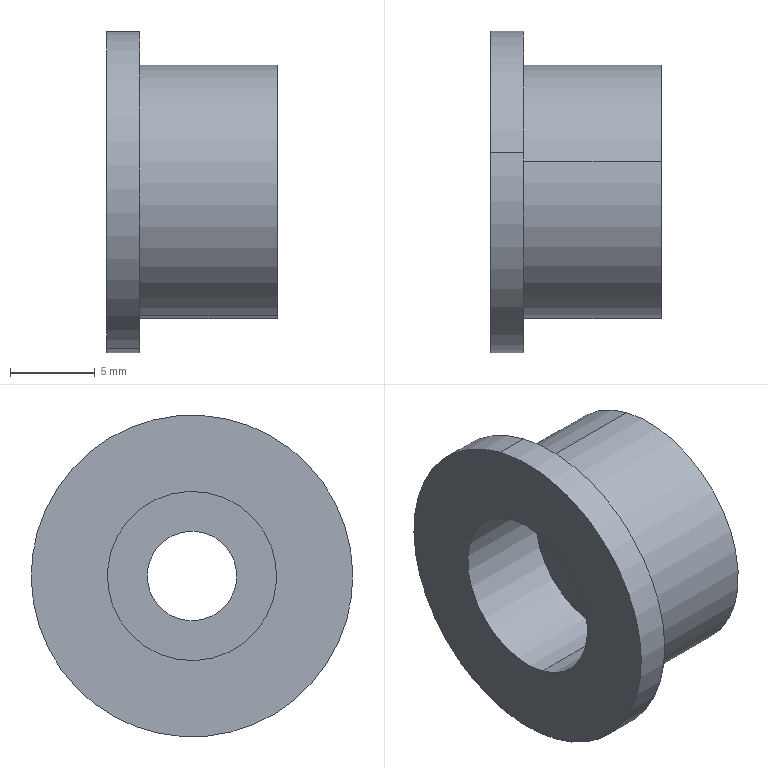Component | SolidWorks | NewDieSet-1_PinDiameter15-3 | 1 solid | 12 faces | box 10.1 x 19 x 19 mm | volume 1448 mm3 | cylinder 8 | plane 4 | commonest cylinder face diameters 10 x2 5.3 x2 19 x2 15 x2
build123d program:
from build123d import *

# Parameters (mm, degrees)
SKETCH1_R                                            = 6
BOSS_EXTRUDE1_DEPTH                                  = 11
SKETCH2_R                                            = 7.5
BOSS_EXTRUDE2_DEPTH                                  = 10.1
SKETCH3_R                                            = 9.5
BOSS_EXTRUDE3_DEPTH                                  = 1.95
HOLE_SIZE_ACCORDING_TO_HEXAGON_SOCKET_HE_D           = 5.3
HOLE_SIZE_ACCORDING_TO_HEXAGON_SOCKET_HE_CBORE_D     = 10
HOLE_SIZE_ACCORDING_TO_HEXAGON_SOCKET_HE_CBORE_DEPTH = 5.7
SKETCH6_R                                            = 6
CUT_EXTRUDE1_DEPTH                                   = 11


with BuildPart() as part:
    # Sketch1 → Boss-Extrude1 (new body)
    with BuildSketch(Plane.XY):
        Circle(SKETCH1_R)
    extrude(amount=BOSS_EXTRUDE1_DEPTH)

    # Sketch2 → Boss-Extrude2 (add)
    with BuildSketch(Plane.XY.offset(11)):
        Circle(SKETCH2_R)
    extrude(amount=BOSS_EXTRUDE2_DEPTH)

    # Sketch3 → Boss-Extrude3 (add)
    with BuildSketch(Plane.XY.offset(21.1)):
        Circle(SKETCH3_R)
    extrude(amount=-BOSS_EXTRUDE3_DEPTH)

    # Hole Size_According to_Hexagon Socket He (through all)
    with Locations(Plane.XY.offset(21.1)):
        with Locations((0, 0)):
            CounterBoreHole(HOLE_SIZE_ACCORDING_TO_HEXAGON_SOCKET_HE_D / 2, HOLE_SIZE_ACCORDING_TO_HEXAGON_SOCKET_HE_CBORE_D / 2, HOLE_SIZE_ACCORDING_TO_HEXAGON_SOCKET_HE_CBORE_DEPTH)

    # Sketch6 → Cut-Extrude1 (cut)
    with BuildSketch(Plane(origin=(0, 0, 0), x_dir=(-1, 0, 0), z_dir=(0, 0, -1))):
        Circle(SKETCH6_R)
    extrude(amount=-CUT_EXTRUDE1_DEPTH, mode=Mode.SUBTRACT)


solid = part.part

# Placed as in the assembly
solid = solid.moved(Location((-245.746, 117.427, 218), (0, -90, 0)))
STEP:
#1=COLOUR_RGB('',0.7922,0.8196,0.9333);
#2=FILL_AREA_STYLE_COLOUR('',#1);
#3=FILL_AREA_STYLE('',(#2));
#4=SURFACE_STYLE_FILL_AREA(#3);
#5=SURFACE_SIDE_STYLE('',(#4));
#6=SURFACE_STYLE_USAGE(.BOTH.,#5);
#7=PRESENTATION_STYLE_ASSIGNMENT((#6));
#8=CARTESIAN_POINT('',(-10.281,4.575,8.392));
#9=VERTEX_POINT('',#8);
#10=CARTESIAN_POINT('',(-10.281,4.671,8.774));
#11=VERTEX_POINT('',#10);
#12=CARTESIAN_POINT('',(-10.281,4.623,8.583));
#13=DIRECTION('',(-1.,-0.,0.));
#14=DIRECTION('',(0.,0.242,0.9703));
#15=AXIS2_PLACEMENT_3D('',#12,#13,#14);
#16=CIRCLE('',#15,0.1969);
#17=EDGE_CURVE('',#9,#11,#16,.T.);
#18=ORIENTED_EDGE('',*,*,#17,.F.);
#19=CARTESIAN_POINT('',(-10.506,4.575,8.392));
#20=VERTEX_POINT('',#19);
#21=CARTESIAN_POINT('',(-10.506,4.575,8.392));
#22=DIRECTION('',(-1.,-0.,0.));
#23=VECTOR('',#22,39.37);
#24=LINE('',#21,#23);
#25=EDGE_CURVE('',#9,#20,#24,.T.);
#26=ORIENTED_EDGE('',*,*,#25,.T.);
#27=CARTESIAN_POINT('',(-10.506,4.671,8.774));
#28=VERTEX_POINT('',#27);
#29=CARTESIAN_POINT('',(-10.506,4.623,8.583));
#30=DIRECTION('',(-1.,-0.,0.));
#31=DIRECTION('',(0.,0.242,0.9703));
#32=AXIS2_PLACEMENT_3D('',#29,#30,#31);
#33=CIRCLE('',#32,0.1969);
#34=EDGE_CURVE('',#20,#28,#33,.T.);
#35=ORIENTED_EDGE('',*,*,#34,.T.);
#36=CARTESIAN_POINT('',(-10.506,4.671,8.774));
#37=DIRECTION('',(-1.,-0.,0.));
#38=VECTOR('',#37,39.37);
#39=LINE('',#36,#38);
#40=EDGE_CURVE('',#11,#28,#39,.T.);
#41=ORIENTED_EDGE('',*,*,#40,.F.);
#42=EDGE_LOOP('',(#18,#26,#35,#41));
#43=FACE_OUTER_BOUND('',#42,.T.);
#44=CARTESIAN_POINT('',(-10.506,4.623,8.583));
#45=DIRECTION('',(-1.,-0.,0.));
#46=DIRECTION('',(0.,0.242,0.9703));
#47=AXIS2_PLACEMENT_3D('',#44,#45,#46);
#48=CYLINDRICAL_SURFACE('',#47,0.1969);
#49=ADVANCED_FACE('',(#43),#48,.F.);
#50=CARTESIAN_POINT('',(-10.108,4.648,8.684));
#51=VERTEX_POINT('',#50);
#52=CARTESIAN_POINT('',(-10.108,4.598,8.481));
#53=VERTEX_POINT('',#52);
#54=CARTESIAN_POINT('',(-10.108,4.623,8.583));
#55=DIRECTION('',(1.,0.,-0.));
#56=DIRECTION('',(0.,0.242,0.9703));
#57=AXIS2_PLACEMENT_3D('',#54,#55,#56);
#58=CIRCLE('',#57,0.1043);
#59=EDGE_CURVE('',#51,#53,#58,.T.);
#60=ORIENTED_EDGE('',*,*,#59,.T.);
#61=CARTESIAN_POINT('',(-10.281,4.598,8.481));
#62=VERTEX_POINT('',#61);
#63=CARTESIAN_POINT('',(-10.506,4.598,8.481));
#64=DIRECTION('',(-1.,-0.,0.));
#65=VECTOR('',#64,39.37);
#66=LINE('',#63,#65);
#67=EDGE_CURVE('',#53,#62,#66,.T.);
#68=ORIENTED_EDGE('',*,*,#67,.T.);
#69=CARTESIAN_POINT('',(-10.281,4.648,8.684));
#70=VERTEX_POINT('',#69);
#71=CARTESIAN_POINT('',(-10.281,4.623,8.583));
#72=DIRECTION('',(-1.,-0.,0.));
#73=DIRECTION('',(0.,0.242,0.9703));
#74=AXIS2_PLACEMENT_3D('',#71,#72,#73);
#75=CIRCLE('',#74,0.1043);
#76=EDGE_CURVE('',#62,#70,#75,.T.);
#77=ORIENTED_EDGE('',*,*,#76,.T.);
#78=CARTESIAN_POINT('',(-10.506,4.648,8.684));
#79=DIRECTION('',(-1.,-0.,0.));
#80=VECTOR('',#79,39.37);
#81=LINE('',#78,#80);
#82=EDGE_CURVE('',#51,#70,#81,.T.);
#83=ORIENTED_EDGE('',*,*,#82,.F.);
#84=EDGE_LOOP('',(#60,#68,#77,#83));
#85=FACE_OUTER_BOUND('',#84,.T.);
#86=CARTESIAN_POINT('',(-10.506,4.623,8.583));
#87=DIRECTION('',(-1.,-0.,0.));
#88=DIRECTION('',(0.,0.242,0.9703));
#89=AXIS2_PLACEMENT_3D('',#86,#87,#88);
#90=CYLINDRICAL_SURFACE('',#89,0.1043);
#91=ADVANCED_FACE('',(#85),#90,.F.);
#92=CARTESIAN_POINT('',(-10.429,4.714,8.946));
#93=VERTEX_POINT('',#92);
#94=CARTESIAN_POINT('',(-10.429,4.533,8.22));
#95=VERTEX_POINT('',#94);
#96=CARTESIAN_POINT('',(-10.429,4.623,8.583));
#97=DIRECTION('',(-1.,-0.,0.));
#98=DIRECTION('',(0.,0.242,0.9703));
#99=AXIS2_PLACEMENT_3D('',#96,#97,#98);
#100=CIRCLE('',#99,0.374);
#101=EDGE_CURVE('',#93,#95,#100,.T.);
#102=ORIENTED_EDGE('',*,*,#101,.T.);
#103=CARTESIAN_POINT('',(-10.506,4.533,8.22));
#104=VERTEX_POINT('',#103);
#105=CARTESIAN_POINT('',(-10.429,4.533,8.22));
#106=DIRECTION('',(-1.,-0.,0.));
#107=VECTOR('',#106,39.37);
#108=LINE('',#105,#107);
#109=EDGE_CURVE('',#95,#104,#108,.T.);
#110=ORIENTED_EDGE('',*,*,#109,.T.);
#111=CARTESIAN_POINT('',(-10.506,4.714,8.946));
#112=VERTEX_POINT('',#111);
#113=CARTESIAN_POINT('',(-10.506,4.623,8.583));
#114=DIRECTION('',(-1.,-0.,0.));
#115=DIRECTION('',(0.,0.242,0.9703));
#116=AXIS2_PLACEMENT_3D('',#113,#114,#115);
#117=CIRCLE('',#116,0.374);
#118=EDGE_CURVE('',#112,#104,#117,.T.);
#119=ORIENTED_EDGE('',*,*,#118,.F.);
#120=CARTESIAN_POINT('',(-10.429,4.714,8.946));
#121=DIRECTION('',(-1.,-0.,0.));
#122=VECTOR('',#121,39.37);
#123=LINE('',#120,#122);
#124=EDGE_CURVE('',#93,#112,#123,.T.);
#125=ORIENTED_EDGE('',*,*,#124,.F.);
#126=EDGE_LOOP('',(#102,#110,#119,#125));
#127=FACE_OUTER_BOUND('',#126,.T.);
#128=CARTESIAN_POINT('',(-10.429,4.623,8.583));
#129=DIRECTION('',(-1.,-0.,0.));
#130=DIRECTION('',(0.,0.242,0.9703));
#131=AXIS2_PLACEMENT_3D('',#128,#129,#130);
#132=CYLINDRICAL_SURFACE('',#131,0.374);
#133=ADVANCED_FACE('',(#127),#132,.T.);
#134=CARTESIAN_POINT('',(-10.429,4.695,8.869));
#135=VERTEX_POINT('',#134);
#136=CARTESIAN_POINT('',(-10.429,4.552,8.296));
#137=VERTEX_POINT('',#136);
#138=CARTESIAN_POINT('',(-10.429,4.623,8.583));
#139=DIRECTION('',(-1.,-0.,0.));
#140=DIRECTION('',(0.,0.242,0.9703));
#141=AXIS2_PLACEMENT_3D('',#138,#139,#140);
#142=CIRCLE('',#141,0.2953);
#143=EDGE_CURVE('',#135,#137,#142,.T.);
#144=ORIENTED_EDGE('',*,*,#143,.F.);
#145=CARTESIAN_POINT('',(-10.108,4.695,8.869));
#146=VERTEX_POINT('',#145);
#147=CARTESIAN_POINT('',(-10.506,4.695,8.869));
#148=DIRECTION('',(1.,0.,-0.));
#149=VECTOR('',#148,39.37);
#150=LINE('',#147,#149);
#151=EDGE_CURVE('',#135,#146,#150,.T.);
#152=ORIENTED_EDGE('',*,*,#151,.T.);
#153=CARTESIAN_POINT('',(-10.108,4.552,8.296));
#154=VERTEX_POINT('',#153);
#155=CARTESIAN_POINT('',(-10.108,4.623,8.583));
#156=DIRECTION('',(-1.,-0.,0.));
#157=DIRECTION('',(0.,0.242,0.9703));
#158=AXIS2_PLACEMENT_3D('',#155,#156,#157);
#159=CIRCLE('',#158,0.2953);
#160=EDGE_CURVE('',#146,#154,#159,.T.);
#161=ORIENTED_EDGE('',*,*,#160,.T.);
#162=CARTESIAN_POINT('',(-10.506,4.552,8.296));
#163=DIRECTION('',(1.,0.,-0.));
#164=VECTOR('',#163,39.37);
#165=LINE('',#162,#164);
#166=EDGE_CURVE('',#137,#154,#165,.T.);
#167=ORIENTED_EDGE('',*,*,#166,.F.);
#168=EDGE_LOOP('',(#144,#152,#161,#167));
#169=FACE_OUTER_BOUND('',#168,.T.);
#170=CARTESIAN_POINT('',(-10.506,4.623,8.583));
#171=DIRECTION('',(1.,0.,-0.));
#172=DIRECTION('',(0.,-0.242,-0.9703));
#173=AXIS2_PLACEMENT_3D('',#170,#171,#172);
#174=CYLINDRICAL_SURFACE('',#173,0.2953);
#175=ADVANCED_FACE('',(#169),#174,.T.);
#176=ORIENTED_EDGE('',*,*,#151,.F.);
#177=CARTESIAN_POINT('',(-10.429,4.623,8.583));
#178=DIRECTION('',(-1.,-0.,0.));
#179=DIRECTION('',(0.,0.242,0.9703));
#180=AXIS2_PLACEMENT_3D('',#177,#178,#179);
#181=CIRCLE('',#180,0.2953);
#182=EDGE_CURVE('',#137,#135,#181,.T.);
#183=ORIENTED_EDGE('',*,*,#182,.F.);
#184=ORIENTED_EDGE('',*,*,#166,.T.);
#185=CARTESIAN_POINT('',(-10.108,4.623,8.583));
#186=DIRECTION('',(-1.,-0.,0.));
#187=DIRECTION('',(0.,0.242,0.9703));
#188=AXIS2_PLACEMENT_3D('',#185,#186,#187);
#189=CIRCLE('',#188,0.2953);
#190=EDGE_CURVE('',#154,#146,#189,.T.);
#191=ORIENTED_EDGE('',*,*,#190,.T.);
#192=EDGE_LOOP('',(#176,#183,#184,#191));
#193=FACE_OUTER_BOUND('',#192,.T.);
#194=CARTESIAN_POINT('',(-10.506,4.623,8.583));
#195=DIRECTION('',(1.,0.,-0.));
#196=DIRECTION('',(0.,-0.242,-0.9703));
#197=AXIS2_PLACEMENT_3D('',#194,#195,#196);
#198=CYLINDRICAL_SURFACE('',#197,0.2953);
#199=ADVANCED_FACE('',(#193),#198,.T.);
#200=ORIENTED_EDGE('',*,*,#190,.F.);
#201=ORIENTED_EDGE('',*,*,#160,.F.);
#202=EDGE_LOOP('',(#200,#201));
#203=FACE_OUTER_BOUND('',#202,.T.);
#204=ORIENTED_EDGE('',*,*,#59,.F.);
#205=CARTESIAN_POINT('',(-10.108,4.623,8.583));
#206=DIRECTION('',(1.,0.,-0.));
#207=DIRECTION('',(0.,0.242,0.9703));
#208=AXIS2_PLACEMENT_3D('',#205,#206,#207);
#209=CIRCLE('',#208,0.1043);
#210=EDGE_CURVE('',#53,#51,#209,.T.);
#211=ORIENTED_EDGE('',*,*,#210,.F.);
#212=EDGE_LOOP('',(#204,#211));
#213=FACE_BOUND('',#212,.T.);
#214=CARTESIAN_POINT('',(-10.108,4.623,8.583));
#215=DIRECTION('',(-1.,0.,0.));
#216=DIRECTION('',(0.,0.242,0.9703));
#217=AXIS2_PLACEMENT_3D('',#214,#215,#216);
#218=PLANE('',#217);
#219=ADVANCED_FACE('',(#203,#213),#218,.F.);
#220=ORIENTED_EDGE('',*,*,#109,.F.);
#221=CARTESIAN_POINT('',(-10.429,4.623,8.583));
#222=DIRECTION('',(-1.,-0.,0.));
#223=DIRECTION('',(0.,0.242,0.9703));
#224=AXIS2_PLACEMENT_3D('',#221,#222,#223);
#225=CIRCLE('',#224,0.374);
#226=EDGE_CURVE('',#95,#93,#225,.T.);
#227=ORIENTED_EDGE('',*,*,#226,.T.);
#228=ORIENTED_EDGE('',*,*,#124,.T.);
#229=CARTESIAN_POINT('',(-10.506,4.623,8.583));
#230=DIRECTION('',(-1.,-0.,0.));
#231=DIRECTION('',(0.,0.242,0.9703));
#232=AXIS2_PLACEMENT_3D('',#229,#230,#231);
#233=CIRCLE('',#232,0.374);
#234=EDGE_CURVE('',#104,#112,#233,.T.);
#235=ORIENTED_EDGE('',*,*,#234,.F.);
#236=EDGE_LOOP('',(#220,#227,#228,#235));
#237=FACE_OUTER_BOUND('',#236,.T.);
#238=CARTESIAN_POINT('',(-10.429,4.623,8.583));
#239=DIRECTION('',(-1.,-0.,0.));
#240=DIRECTION('',(0.,0.242,0.9703));
#241=AXIS2_PLACEMENT_3D('',#238,#239,#240);
#242=CYLINDRICAL_SURFACE('',#241,0.374);
#243=ADVANCED_FACE('',(#237),#242,.T.);
#244=ORIENTED_EDGE('',*,*,#182,.T.);
#245=ORIENTED_EDGE('',*,*,#143,.T.);
#246=EDGE_LOOP('',(#244,#245));
#247=FACE_BOUND('',#246,.T.);
#248=ORIENTED_EDGE('',*,*,#101,.F.);
#249=ORIENTED_EDGE('',*,*,#226,.F.);
#250=EDGE_LOOP('',(#248,#249));
#251=FACE_OUTER_BOUND('',#250,.T.);
#252=CARTESIAN_POINT('',(-10.429,4.623,8.583));
#253=DIRECTION('',(-1.,0.,0.));
#254=DIRECTION('',(0.,0.242,0.9703));
#255=AXIS2_PLACEMENT_3D('',#252,#253,#254);
#256=PLANE('',#255);
#257=ADVANCED_FACE('',(#247,#251),#256,.F.);
#258=CARTESIAN_POINT('',(-10.506,4.623,8.583));
#259=DIRECTION('',(-1.,-0.,0.));
#260=DIRECTION('',(0.,0.242,0.9703));
#261=AXIS2_PLACEMENT_3D('',#258,#259,#260);
#262=CIRCLE('',#261,0.1969);
#263=EDGE_CURVE('',#28,#20,#262,.T.);
#264=ORIENTED_EDGE('',*,*,#263,.F.);
#265=ORIENTED_EDGE('',*,*,#34,.F.);
#266=EDGE_LOOP('',(#264,#265));
#267=FACE_BOUND('',#266,.T.);
#268=ORIENTED_EDGE('',*,*,#118,.T.);
#269=ORIENTED_EDGE('',*,*,#234,.T.);
#270=EDGE_LOOP('',(#268,#269));
#271=FACE_OUTER_BOUND('',#270,.T.);
#272=CARTESIAN_POINT('',(-10.506,4.623,8.583));
#273=DIRECTION('',(-1.,0.,0.));
#274=DIRECTION('',(0.,0.242,0.9703));
#275=AXIS2_PLACEMENT_3D('',#272,#273,#274);
#276=PLANE('',#275);
#277=ADVANCED_FACE('',(#267,#271),#276,.T.);
#278=ORIENTED_EDGE('',*,*,#67,.F.);
#279=ORIENTED_EDGE('',*,*,#210,.T.);
#280=ORIENTED_EDGE('',*,*,#82,.T.);
#281=CARTESIAN_POINT('',(-10.281,4.623,8.583));
#282=DIRECTION('',(-1.,-0.,0.));
#283=DIRECTION('',(0.,0.242,0.9703));
#284=AXIS2_PLACEMENT_3D('',#281,#282,#283);
#285=CIRCLE('',#284,0.1043);
#286=EDGE_CURVE('',#70,#62,#285,.T.);
#287=ORIENTED_EDGE('',*,*,#286,.T.);
#288=EDGE_LOOP('',(#278,#279,#280,#287));
#289=FACE_OUTER_BOUND('',#288,.T.);
#290=CARTESIAN_POINT('',(-10.506,4.623,8.583));
#291=DIRECTION('',(-1.,-0.,0.));
#292=DIRECTION('',(0.,0.242,0.9703));
#293=AXIS2_PLACEMENT_3D('',#290,#291,#292);
#294=CYLINDRICAL_SURFACE('',#293,0.1043);
#295=ADVANCED_FACE('',(#289),#294,.F.);
#296=ORIENTED_EDGE('',*,*,#286,.F.);
#297=ORIENTED_EDGE('',*,*,#76,.F.);
#298=EDGE_LOOP('',(#296,#297));
#299=FACE_BOUND('',#298,.T.);
#300=CARTESIAN_POINT('',(-10.281,4.623,8.583));
#301=DIRECTION('',(-1.,-0.,0.));
#302=DIRECTION('',(0.,0.242,0.9703));
#303=AXIS2_PLACEMENT_3D('',#300,#301,#302);
#304=CIRCLE('',#303,0.1969);
#305=EDGE_CURVE('',#11,#9,#304,.T.);
#306=ORIENTED_EDGE('',*,*,#305,.T.);
#307=ORIENTED_EDGE('',*,*,#17,.T.);
#308=EDGE_LOOP('',(#306,#307));
#309=FACE_OUTER_BOUND('',#308,.T.);
#310=CARTESIAN_POINT('',(-10.281,4.648,8.684));
#311=DIRECTION('',(1.,-0.,-0.));
#312=DIRECTION('',(-0.,-0.242,-0.9703));
#313=AXIS2_PLACEMENT_3D('',#310,#311,#312);
#314=PLANE('',#313);
#315=ADVANCED_FACE('',(#299,#309),#314,.F.);
#316=ORIENTED_EDGE('',*,*,#25,.F.);
#317=ORIENTED_EDGE('',*,*,#305,.F.);
#318=ORIENTED_EDGE('',*,*,#40,.T.);
#319=ORIENTED_EDGE('',*,*,#263,.T.);
#320=EDGE_LOOP('',(#316,#317,#318,#319));
#321=FACE_OUTER_BOUND('',#320,.T.);
#322=CARTESIAN_POINT('',(-10.506,4.623,8.583));
#323=DIRECTION('',(-1.,-0.,0.));
#324=DIRECTION('',(0.,0.242,0.9703));
#325=AXIS2_PLACEMENT_3D('',#322,#323,#324);
#326=CYLINDRICAL_SURFACE('',#325,0.1969);
#327=ADVANCED_FACE('',(#321),#326,.F.);
#328=CLOSED_SHELL('',(#49,#91,#133,#175,#199,#219,#243,#257,#277,#295,#315,#327));
#329=MANIFOLD_SOLID_BREP('',#328);
#330=STYLED_ITEM('',(#7),#329);
#331=(LENGTH_UNIT()NAMED_UNIT(*)SI_UNIT($,.METRE.));
#332=LENGTH_MEASURE_WITH_UNIT(LENGTH_MEASURE(0.0254),#331);
#333=DIMENSIONAL_EXPONENTS(1.,0.,0.,0.,0.,0.,0.);
#334=(CONVERSION_BASED_UNIT('',#332)LENGTH_UNIT()NAMED_UNIT(#333));
#335=UNCERTAINTY_MEASURE_WITH_UNIT(LENGTH_MEASURE(0.00001),#334,'','');
#336=(NAMED_UNIT(*)PLANE_ANGLE_UNIT()SI_UNIT($,.RADIAN.));
#337=(NAMED_UNIT(*)SI_UNIT($,.STERADIAN.)SOLID_ANGLE_UNIT());
#338=(GEOMETRIC_REPRESENTATION_CONTEXT(3)GLOBAL_UNCERTAINTY_ASSIGNED_CONTEXT((#335))GLOBAL_UNIT_ASSIGNED_CONTEXT((#334,#336,#337))REPRESENTATION_CONTEXT('',''));
#339=MECHANICAL_DESIGN_GEOMETRIC_PRESENTATION_REPRESENTATION('',(#330),#338);
#340=CARTESIAN_POINT('',(0.,0.,0.));
#341=DIRECTION('',(0.,0.,1.));
#342=DIRECTION('',(1.,0.,0.));
#343=AXIS2_PLACEMENT_3D('',#340,#341,#342);
#344=(LENGTH_UNIT()NAMED_UNIT(*)SI_UNIT($,.METRE.));
#345=LENGTH_MEASURE_WITH_UNIT(LENGTH_MEASURE(0.0254),#344);
#346=DIMENSIONAL_EXPONENTS(1.,0.,0.,0.,0.,0.,0.);
#347=(CONVERSION_BASED_UNIT('',#345)LENGTH_UNIT()NAMED_UNIT(#346));
#348=UNCERTAINTY_MEASURE_WITH_UNIT(LENGTH_MEASURE(0.00001),#347,'','');
#349=(NAMED_UNIT(*)PLANE_ANGLE_UNIT()SI_UNIT($,.RADIAN.));
#350=(NAMED_UNIT(*)SI_UNIT($,.STERADIAN.)SOLID_ANGLE_UNIT());
#351=(GEOMETRIC_REPRESENTATION_CONTEXT(3)GLOBAL_UNCERTAINTY_ASSIGNED_CONTEXT((#348))GLOBAL_UNIT_ASSIGNED_CONTEXT((#347,#349,#350))REPRESENTATION_CONTEXT('',''));
#352=ADVANCED_BREP_SHAPE_REPRESENTATION('',(#329,#343),#351);
#353=PRESENTATION_LAYER_ASSIGNMENT('','',(#330));